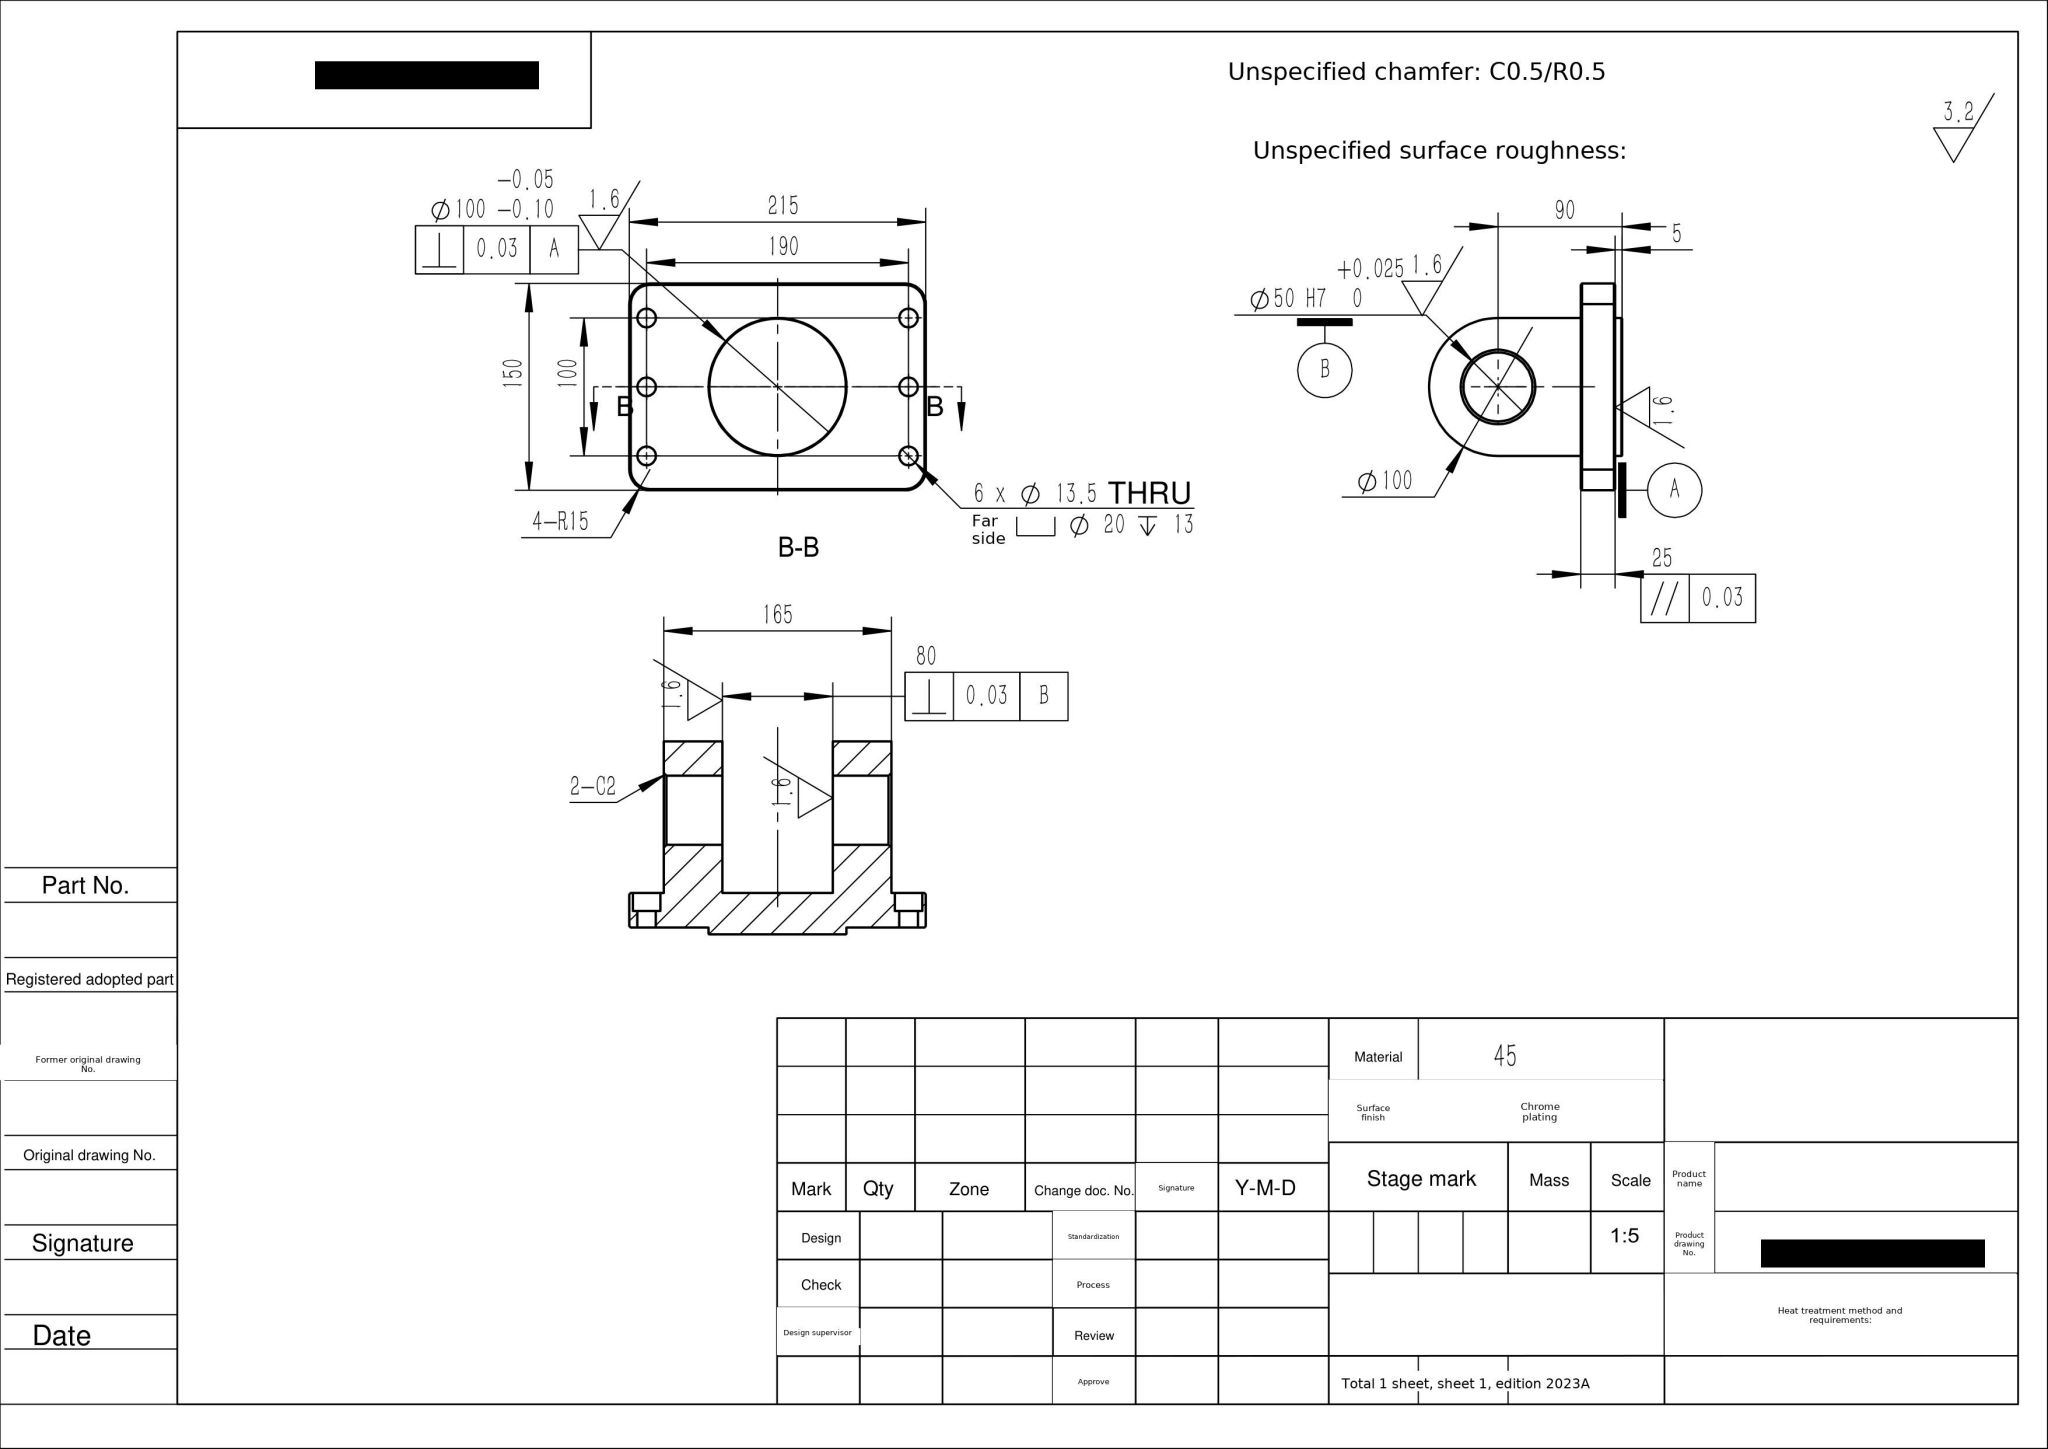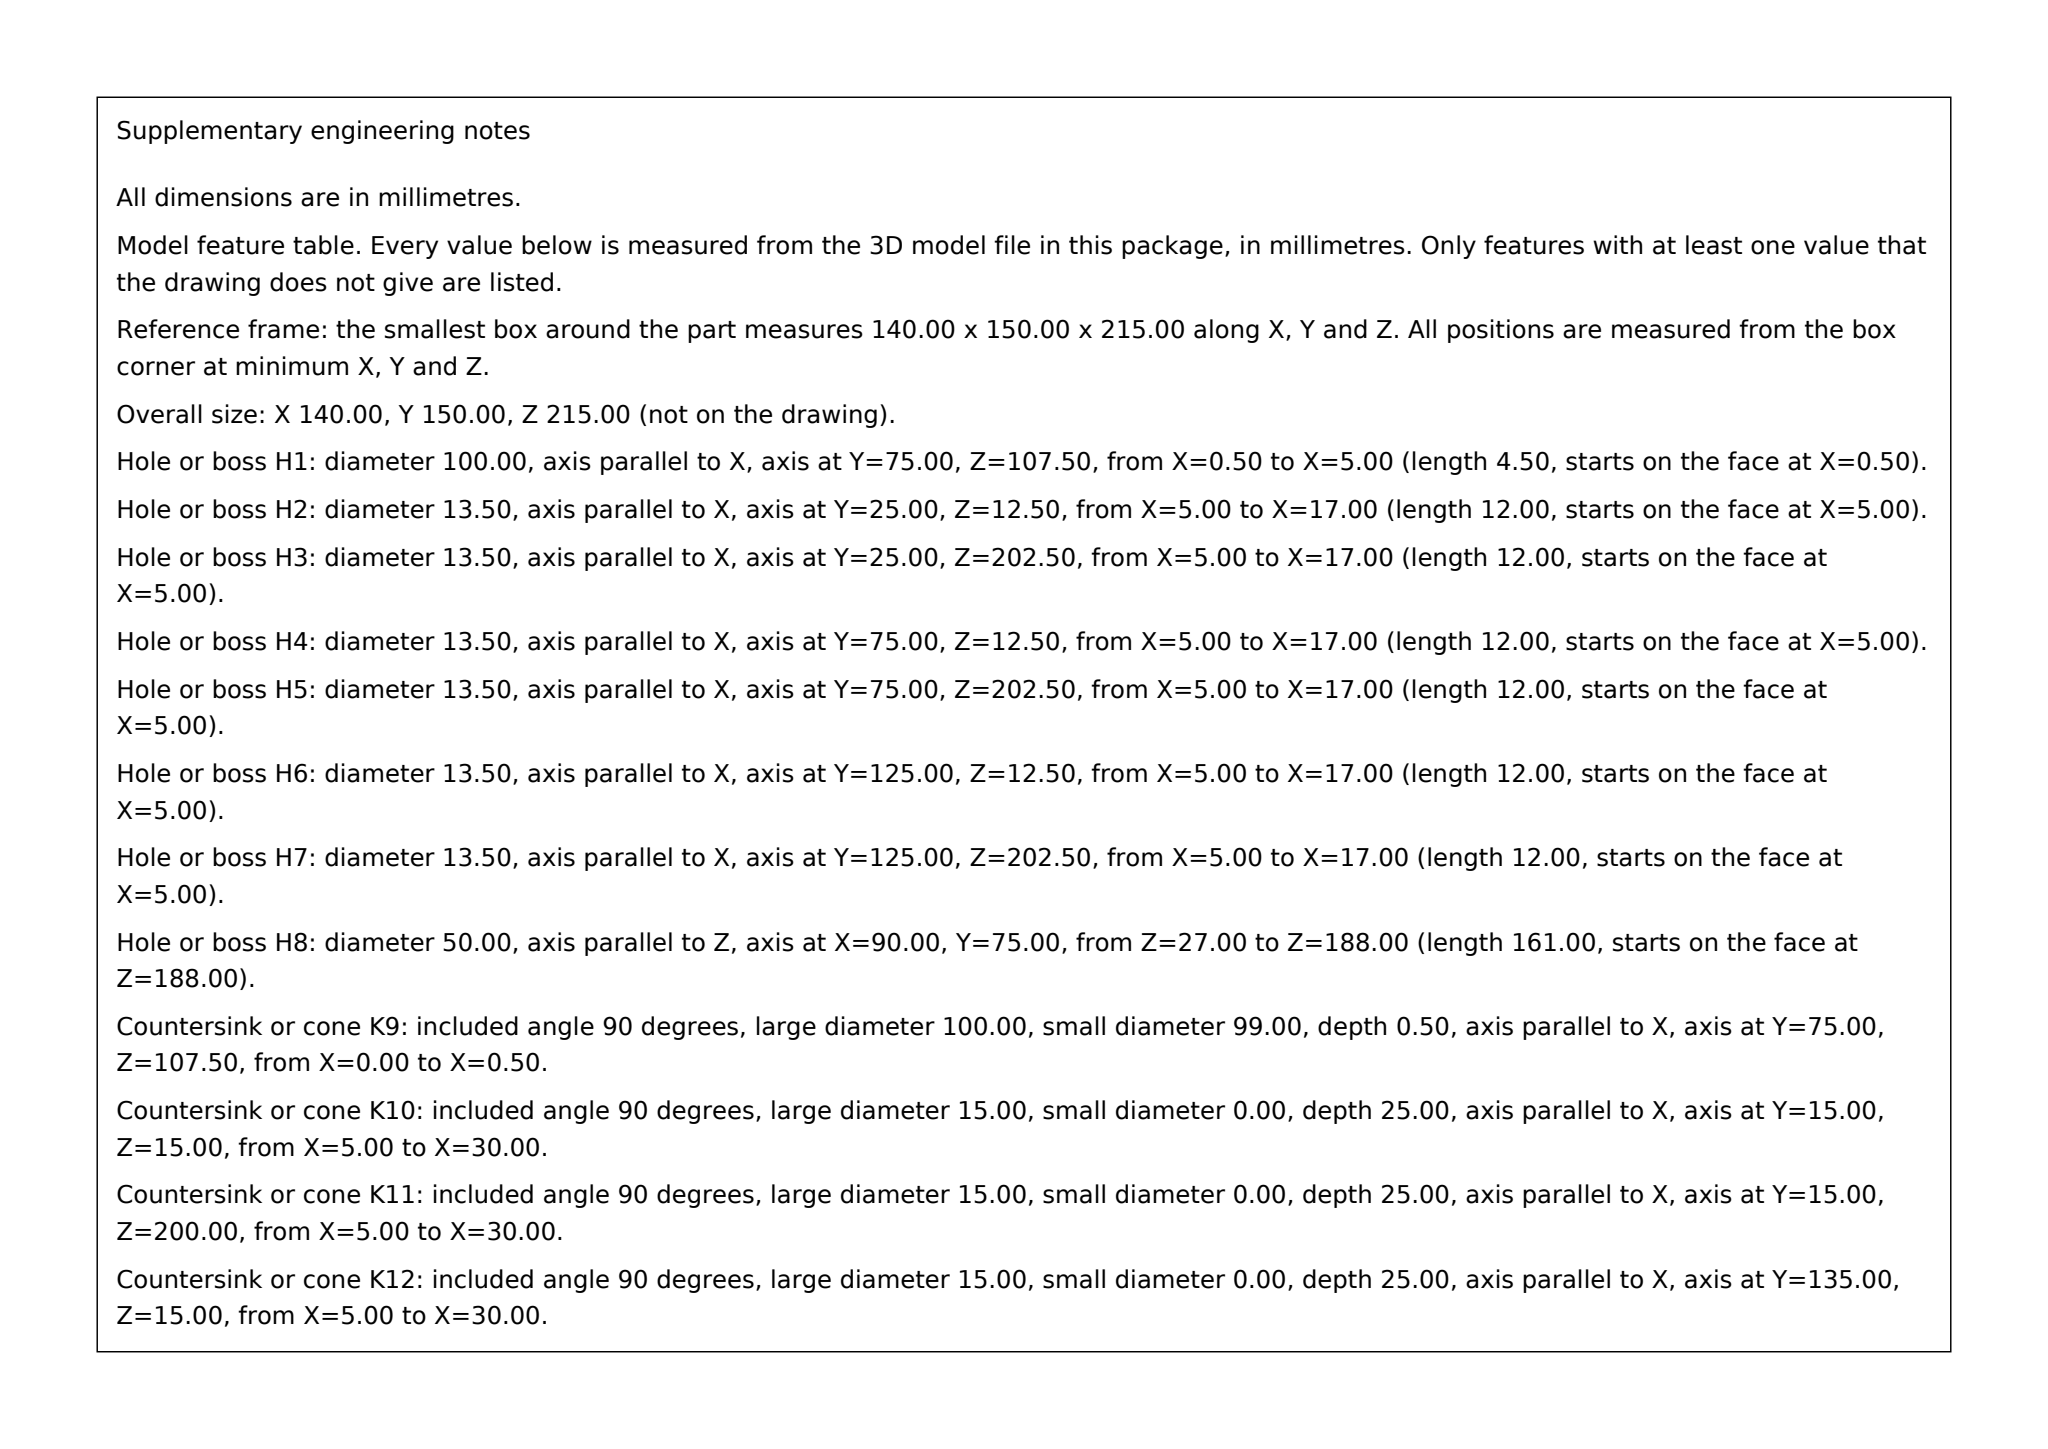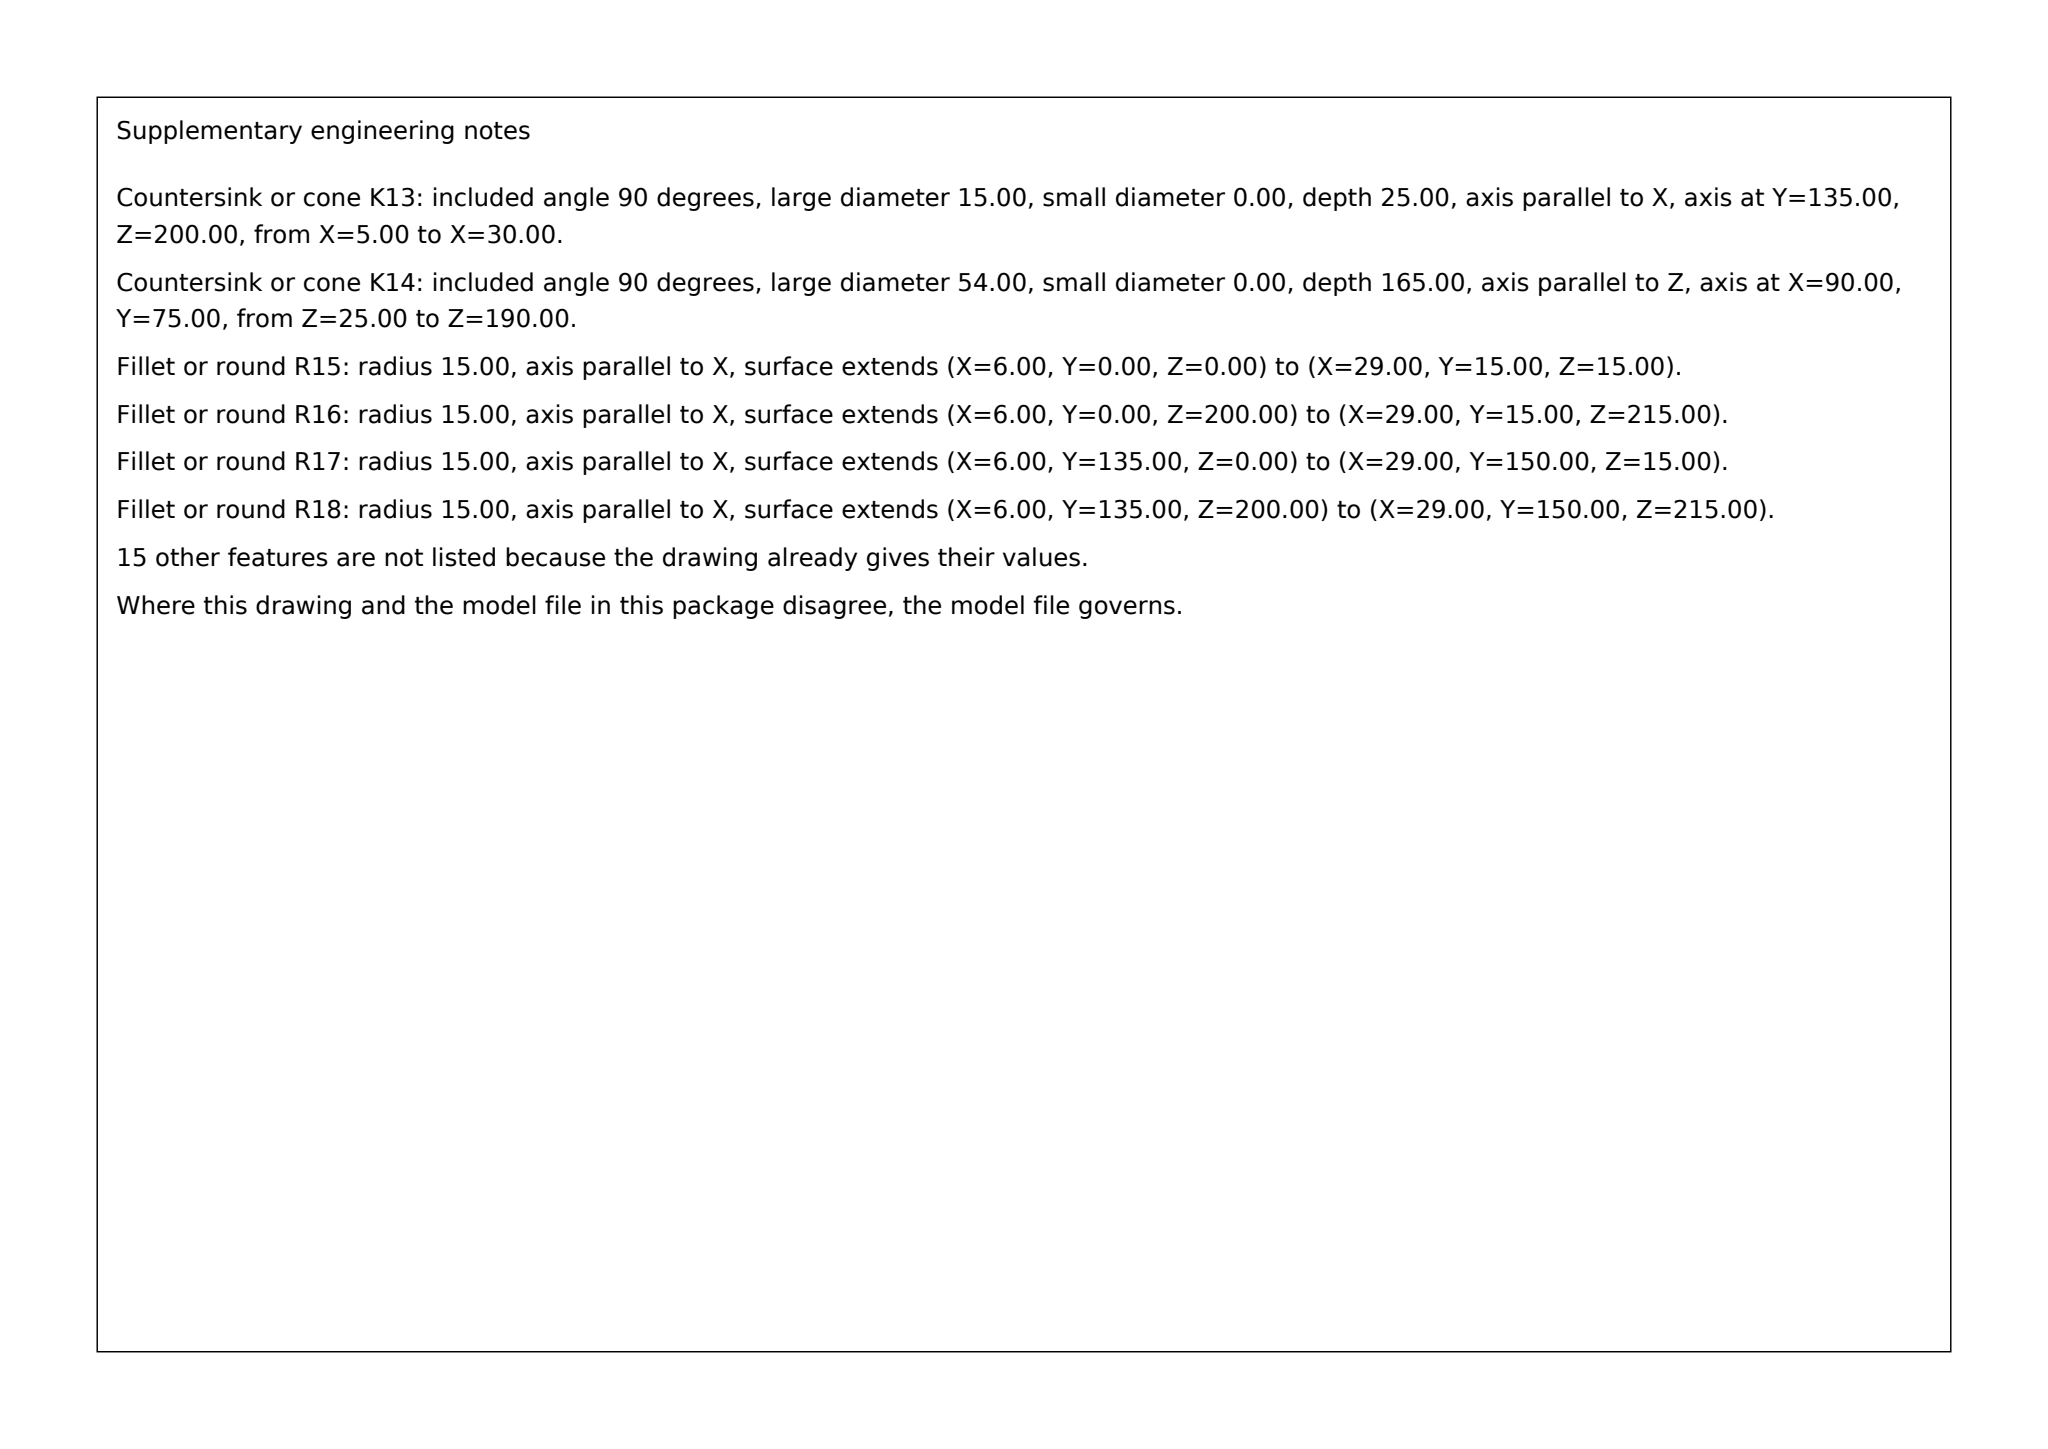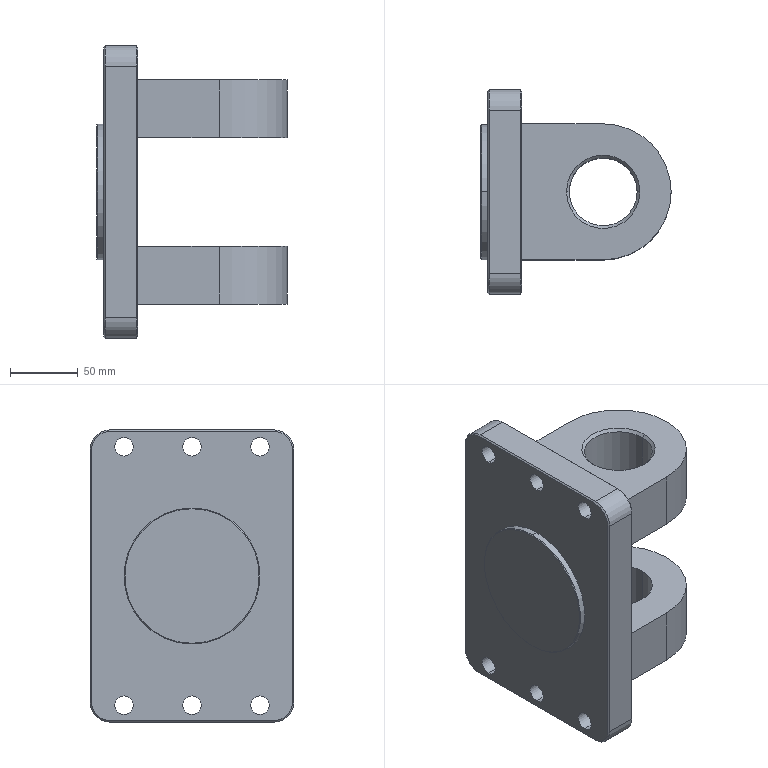Part | SolidWorks | mm | material 45 | 1 solid | 81 faces | box 140 x 150 x 215 mm | volume 1481392 mm3 | cylinder 38 | plane 29 | cone 14 | commonest cylinder face diameters 20 x12 13.5 x12 100 x6 50 x4 30 x4